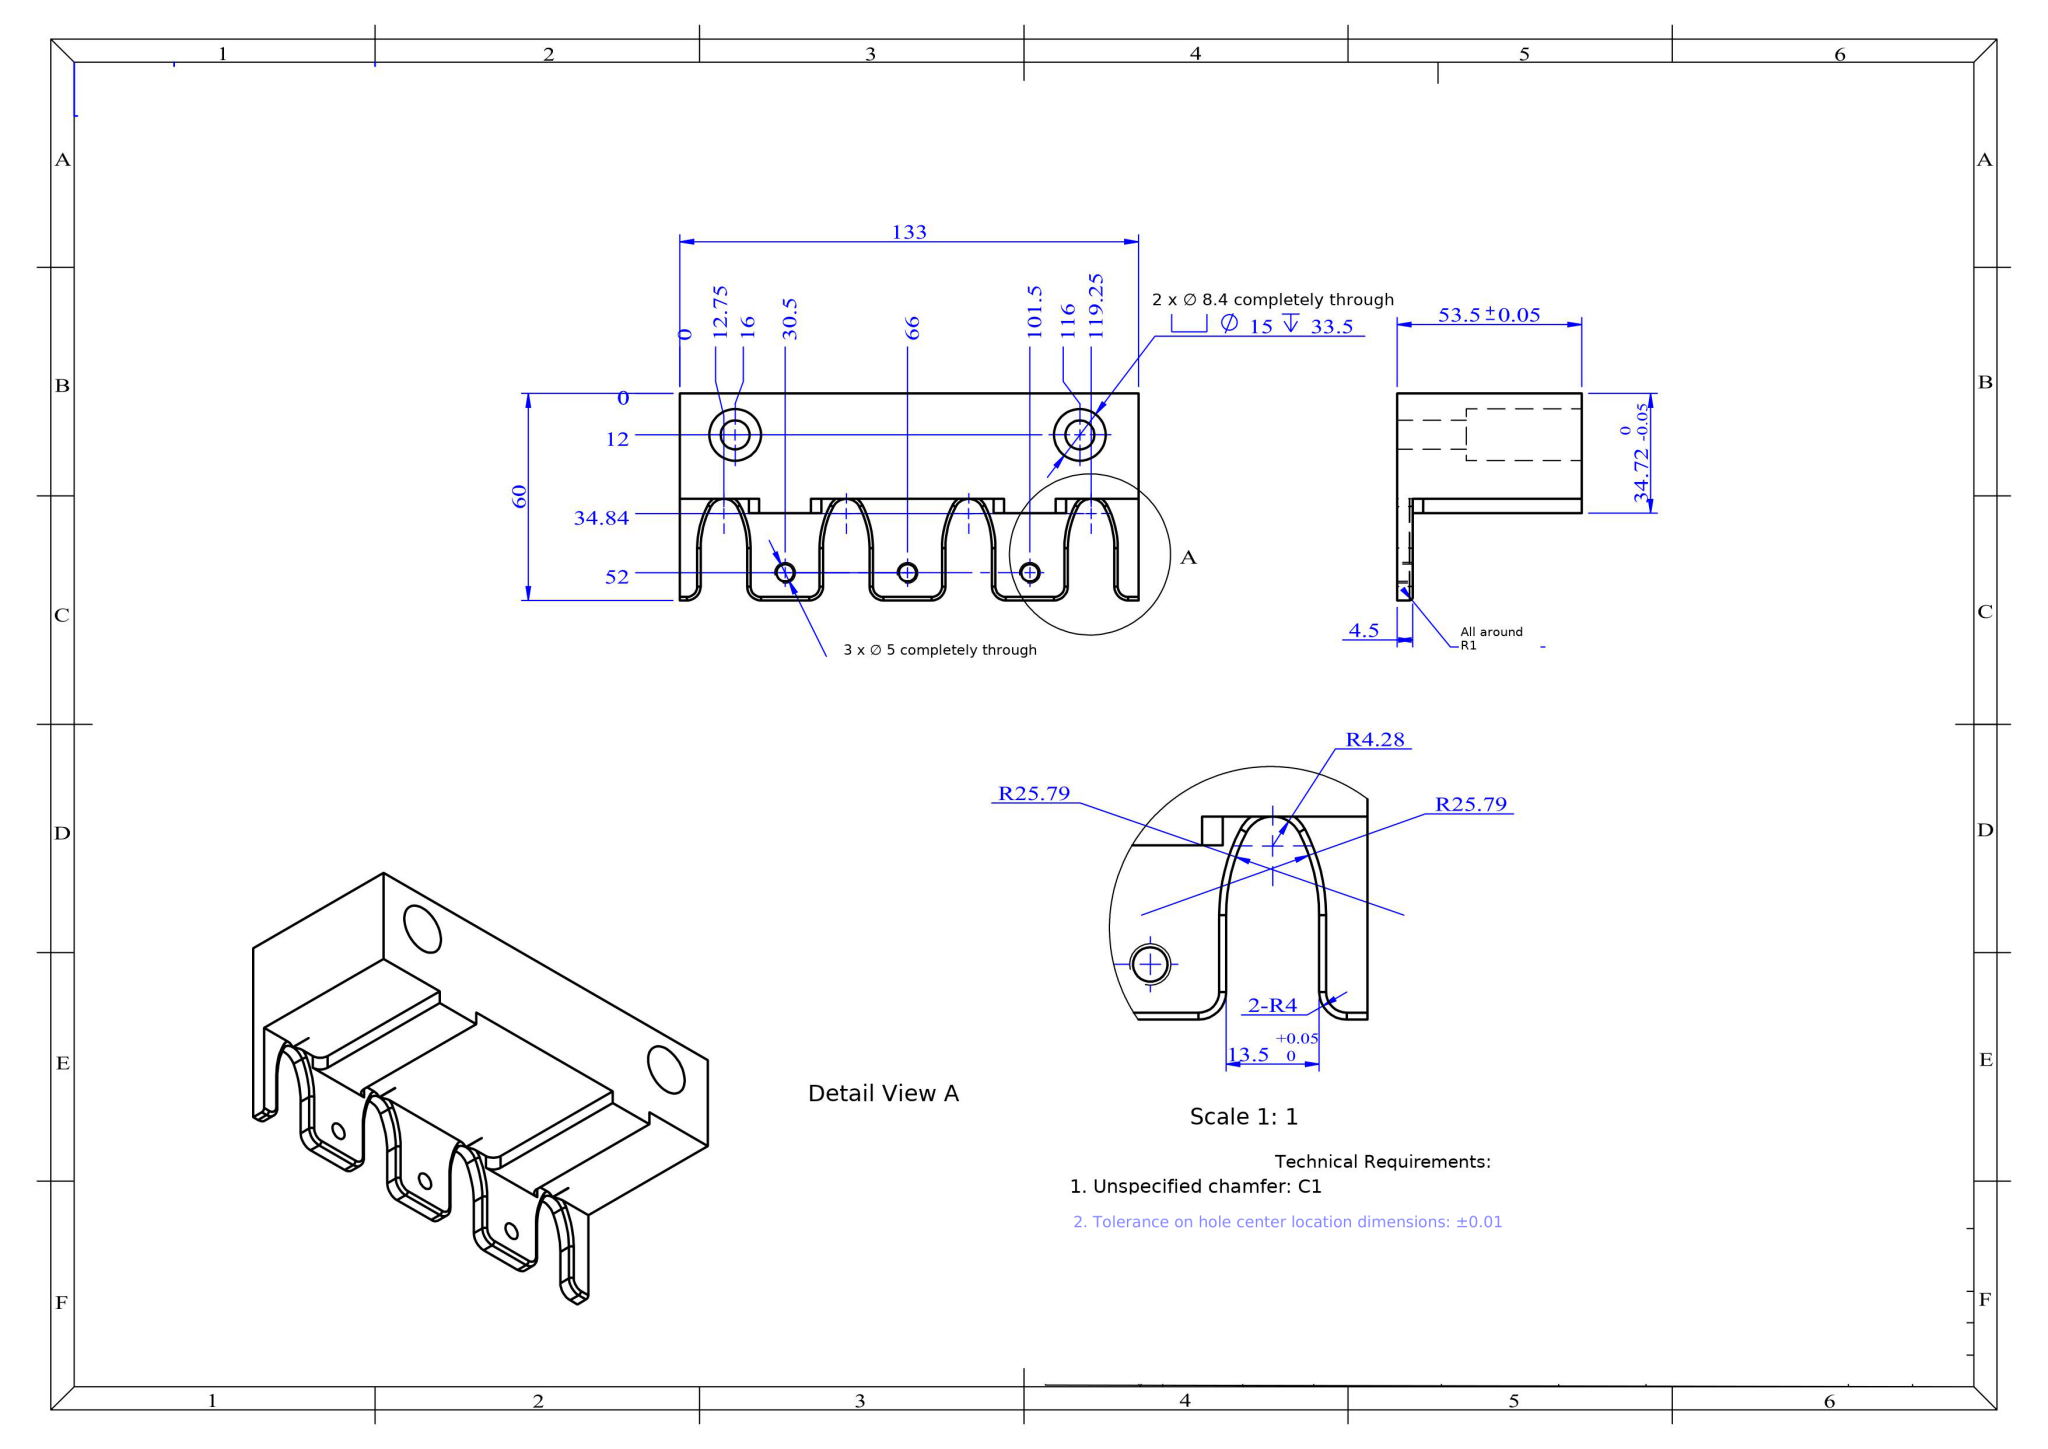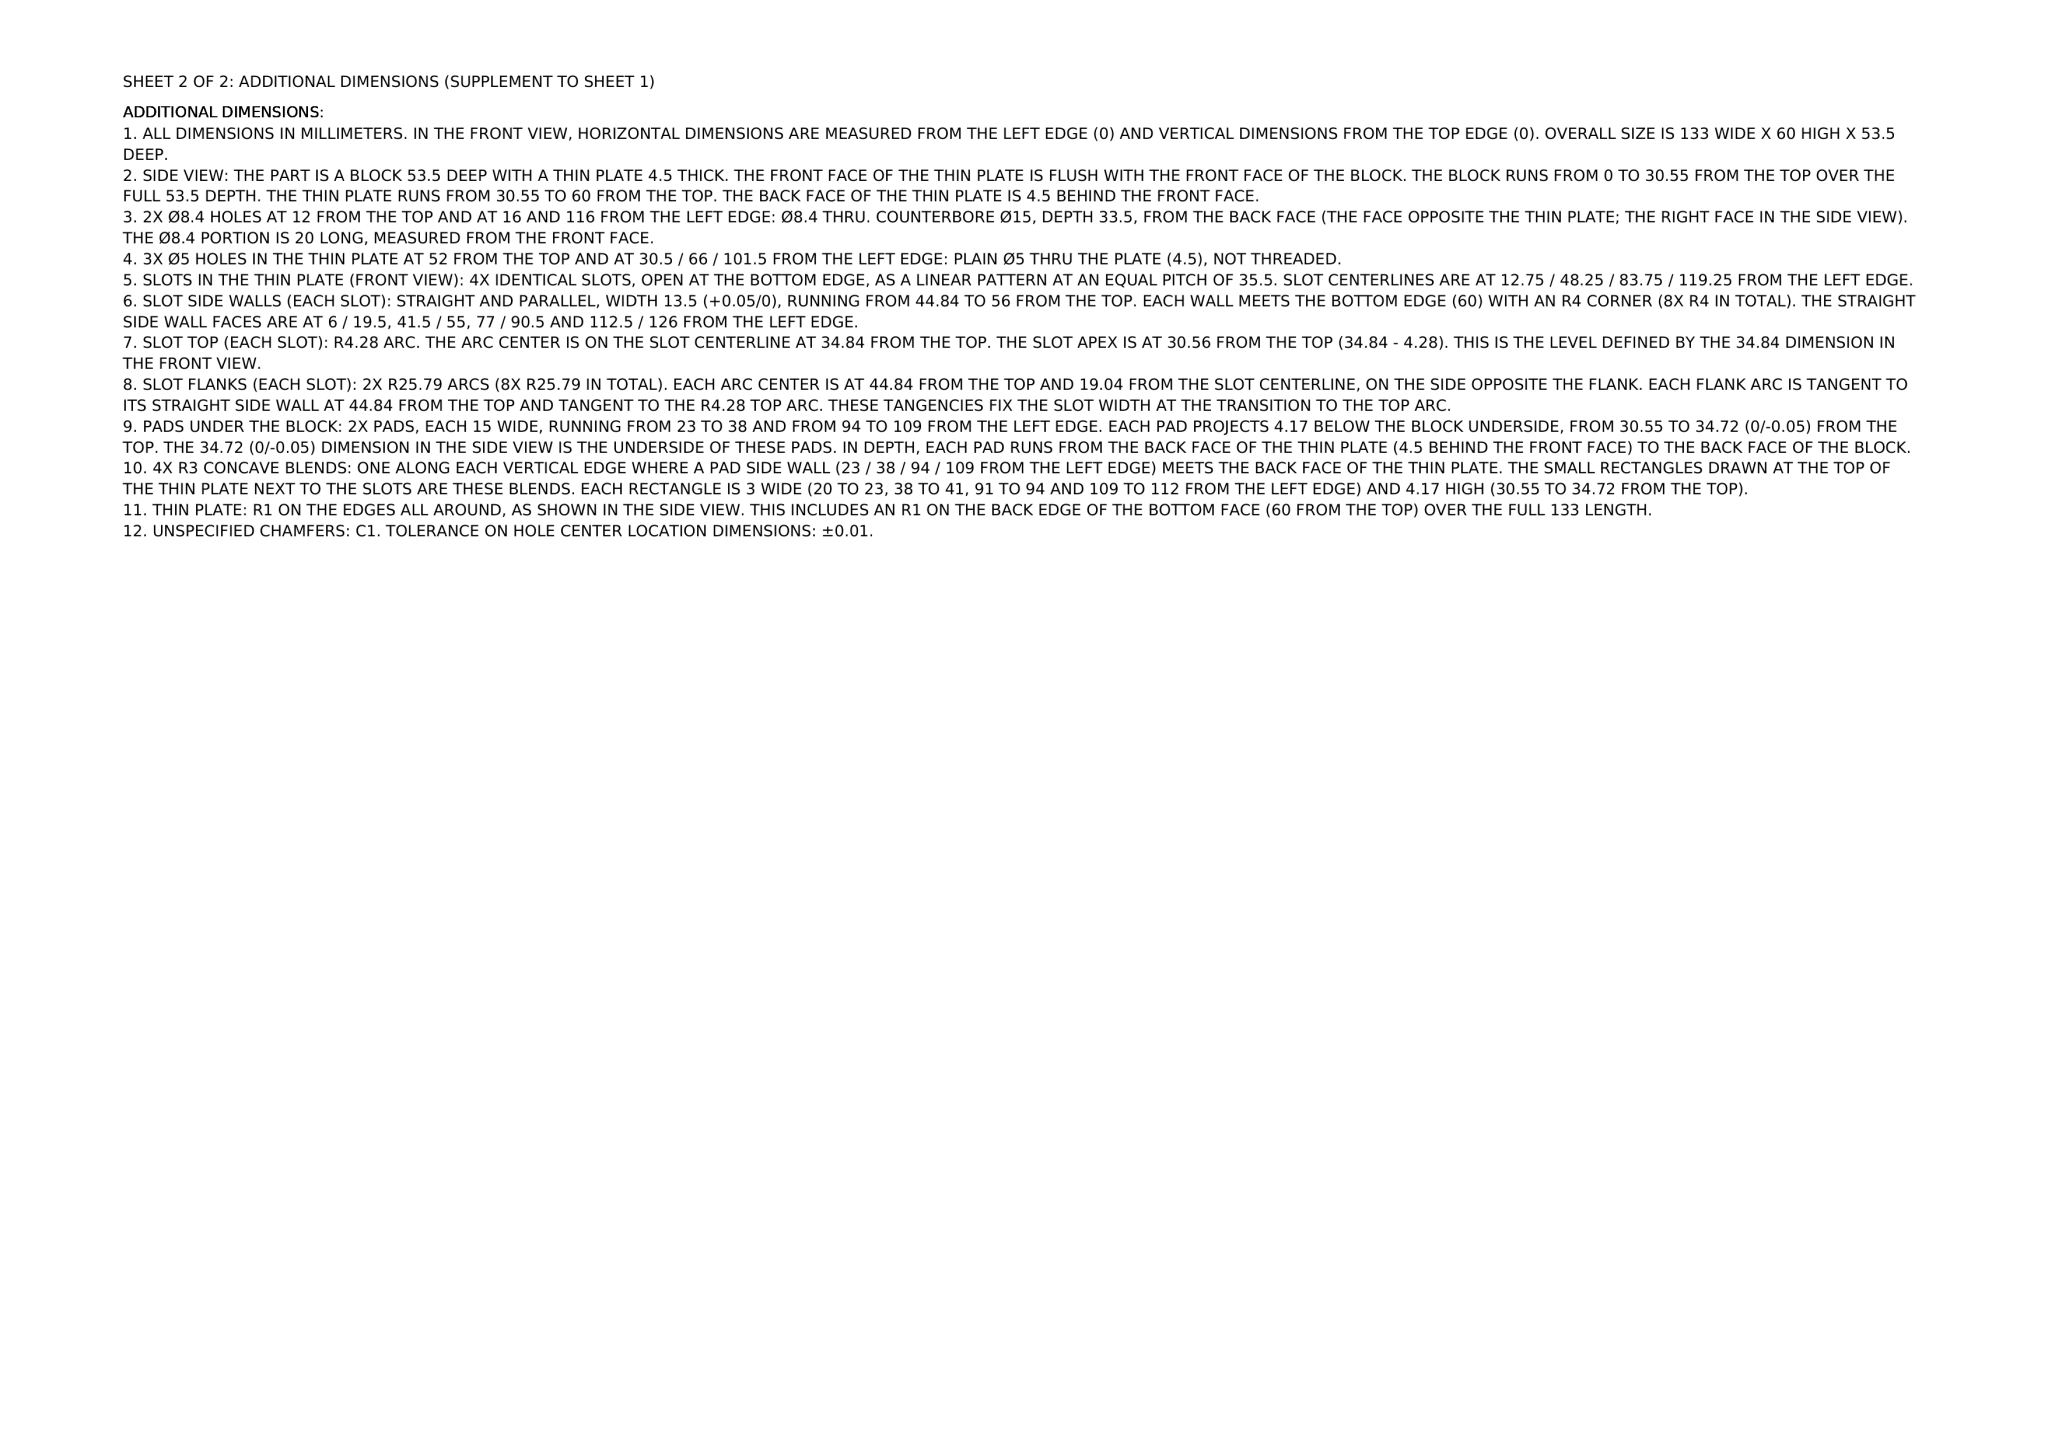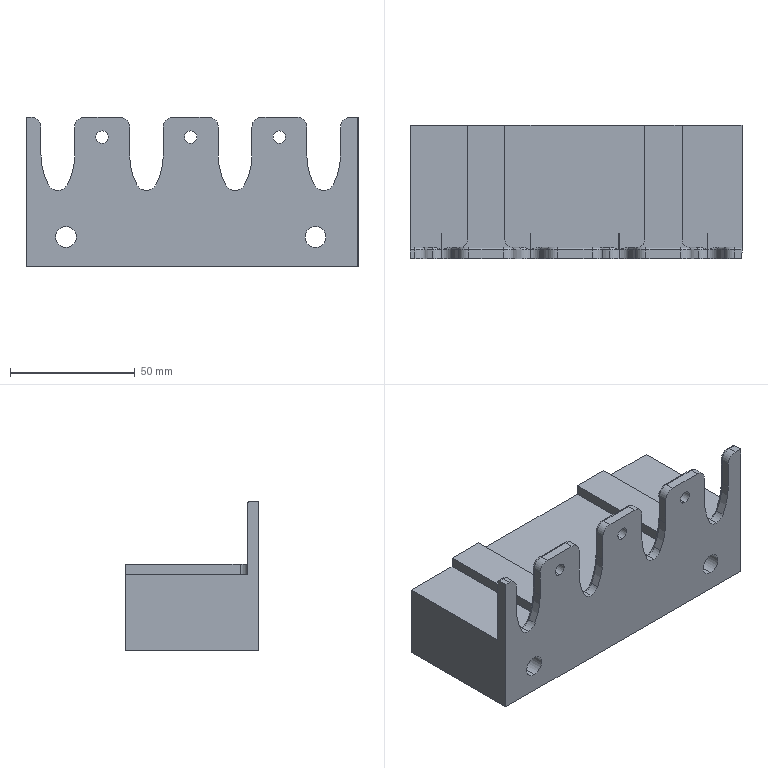Part | NX | mm | 1 solid | 113 faces | box 133 x 53.5 x 60 mm | volume 220266 mm3 | cylinder 55 | plane 34 | torus 24 | commonest cylinder face diameters 2 x13 8.564 x8 51.575 x8 8 x8 5 x6 15 x4 8.4 x4 6 x4